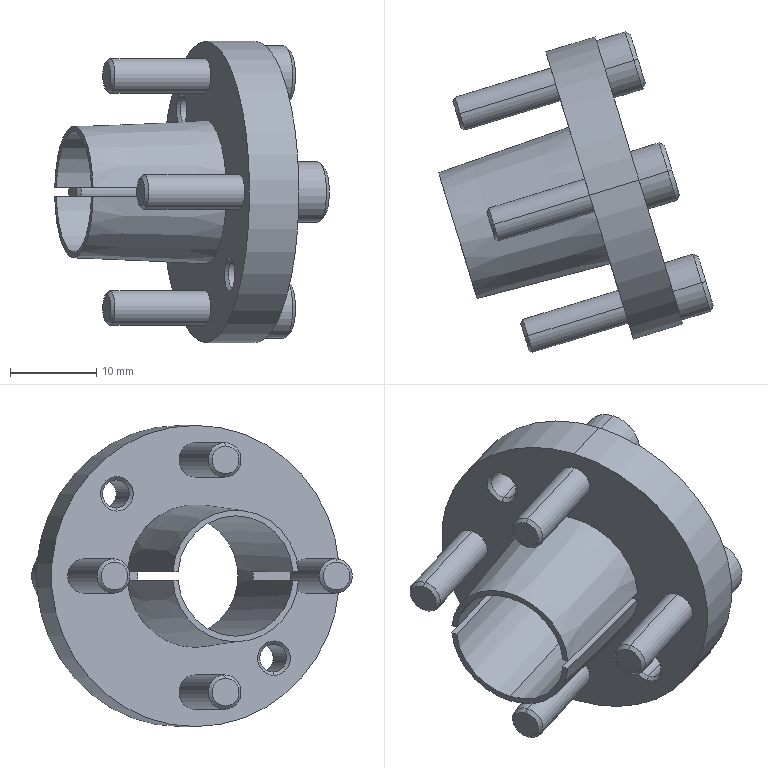Component | SolidWorks | v1ZHXTPTLA36P5M100_E_14SB1-1_v1ZHXT14SB1-1 | 1 solid | 131 faces | box 31.91 x 37.25 x 35 mm | volume 6607 mm3 | plane 64 | cone 43 | cylinder 24 | commonest cylinder face diameters 7 x8 4 x8 3.242 x4 35 x2 14 x2